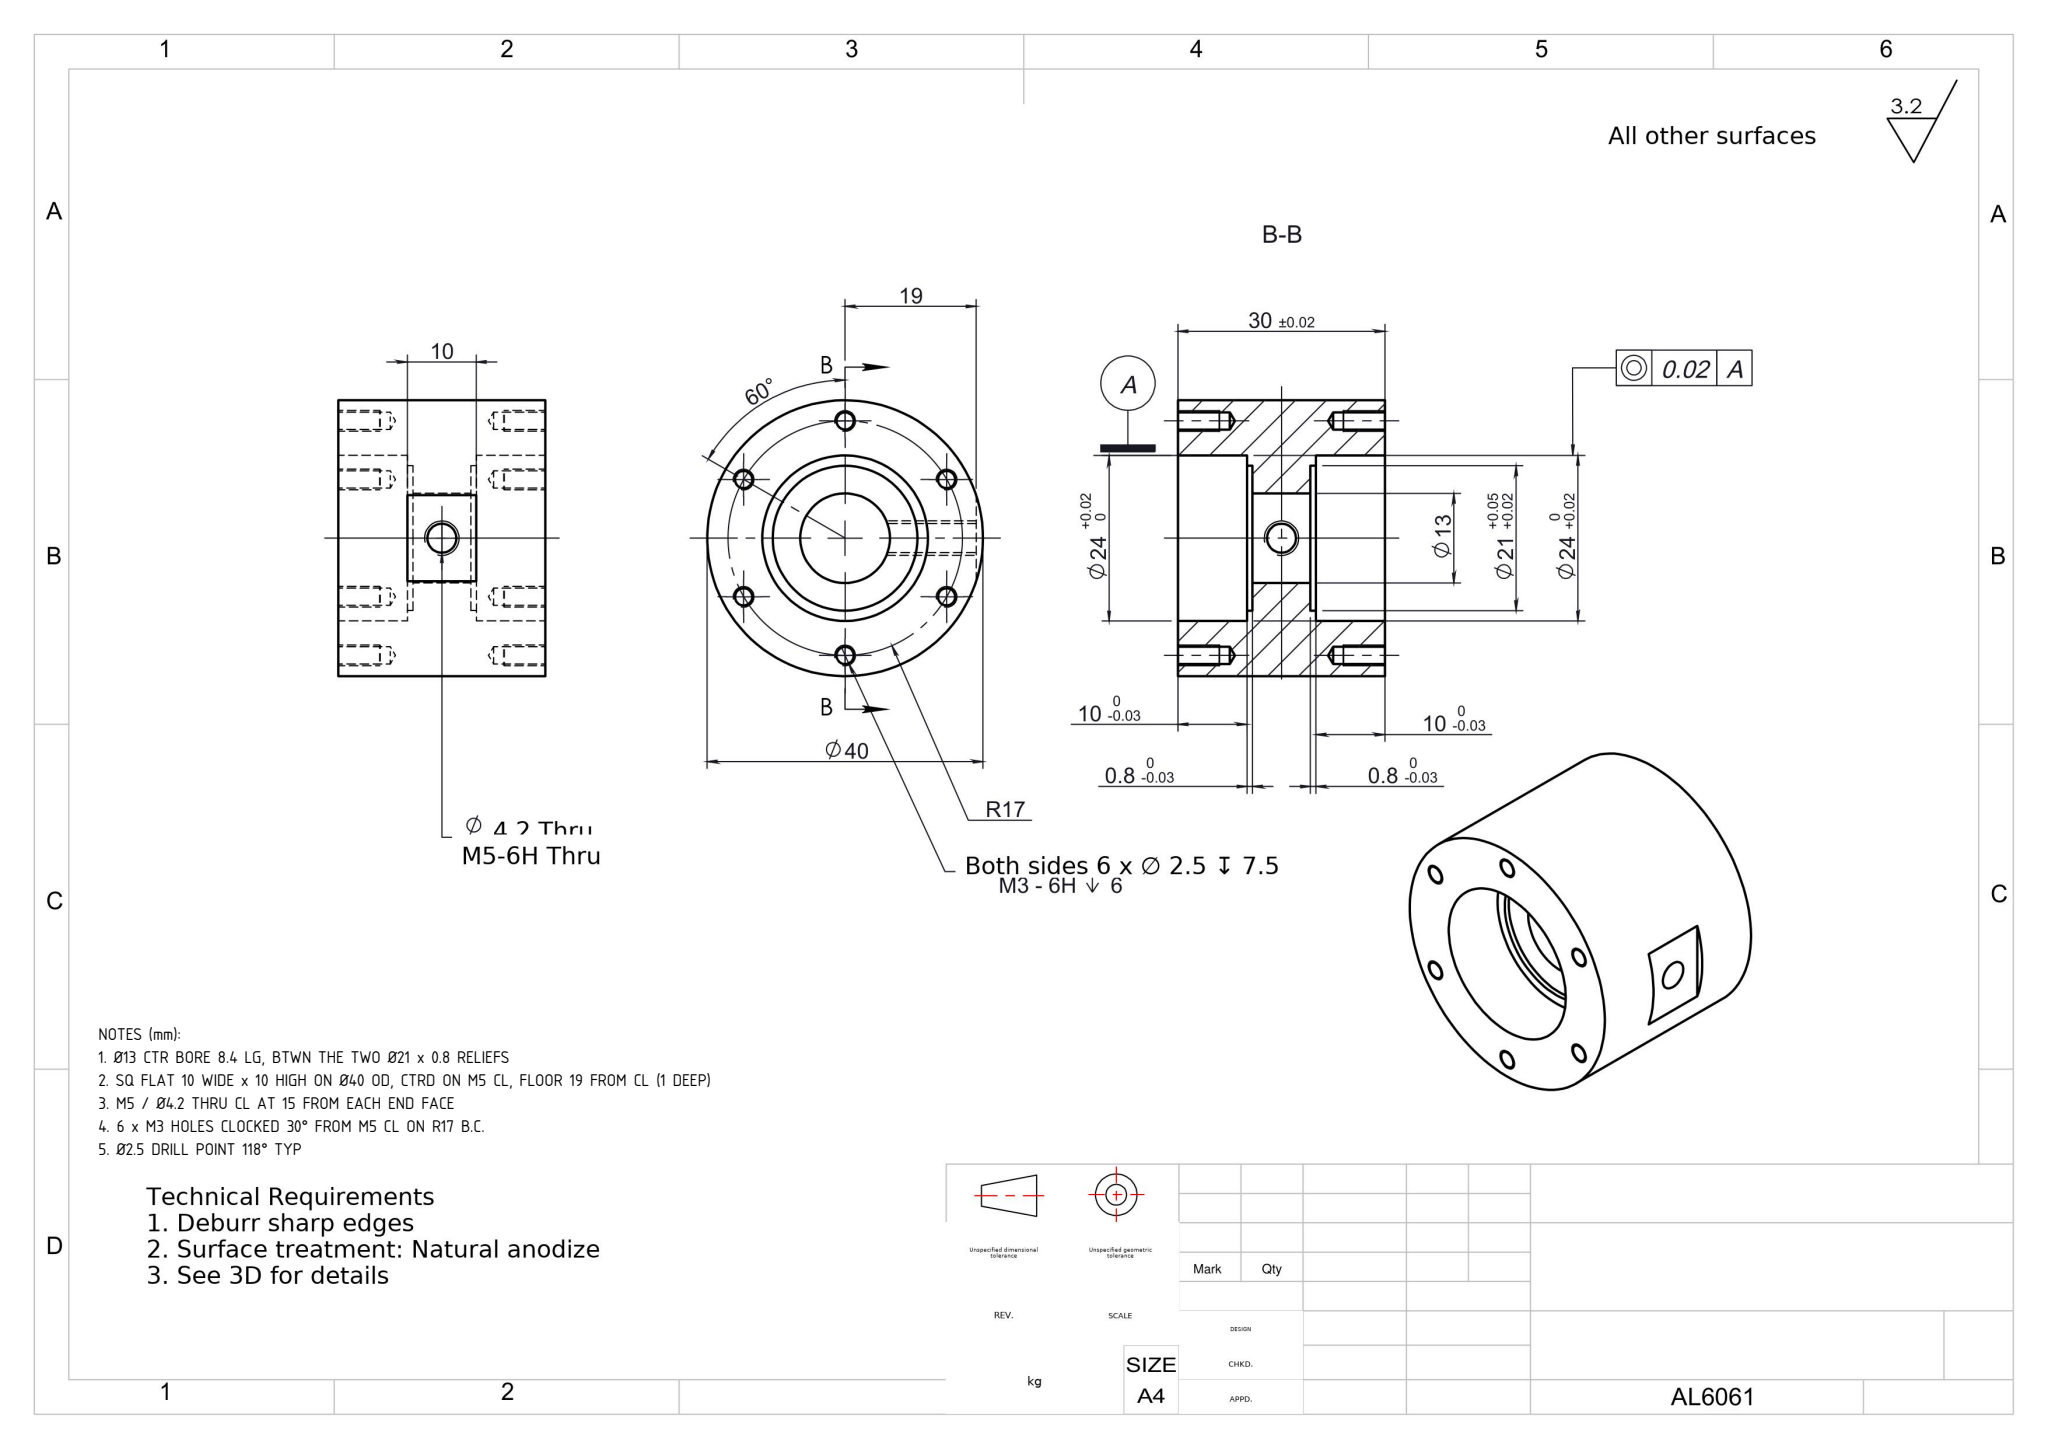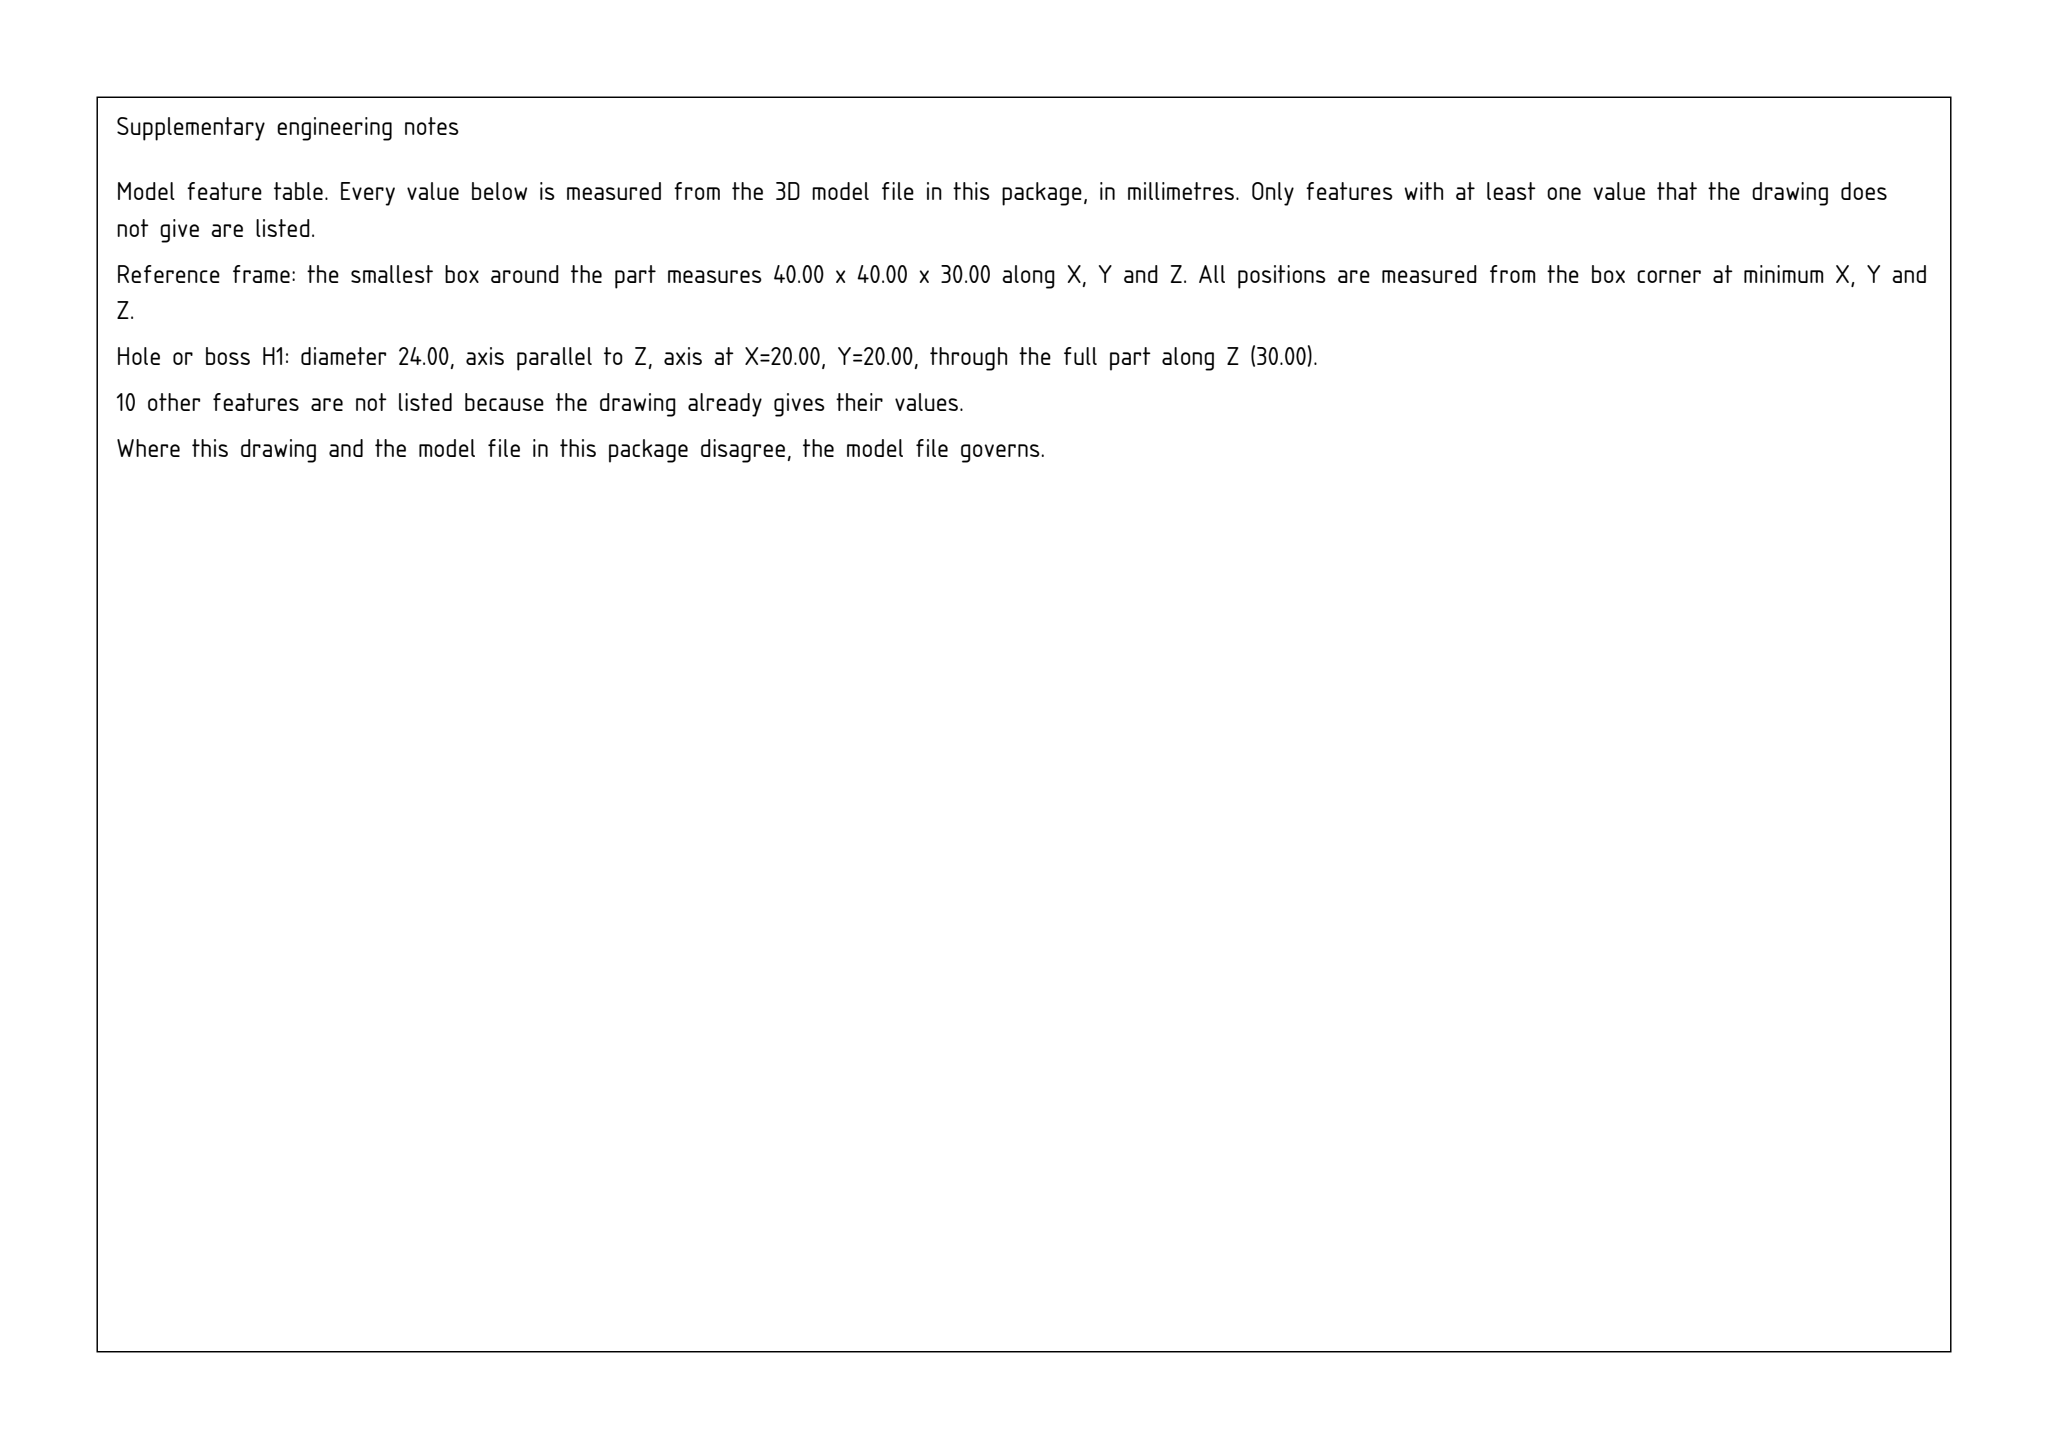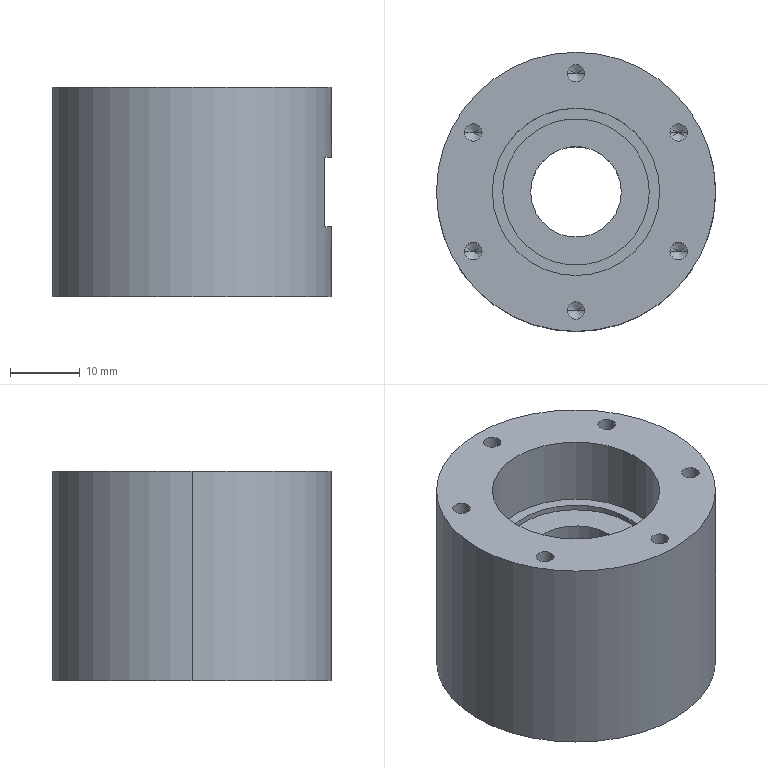Part | SolidWorks | mm | 1 solid | 71 faces | box 40 x 40 x 30 mm | volume 26268 mm3 | cylinder 38 | cone 24 | plane 9 | commonest cylinder face diameters 2.5 x24 21 x4 24 x4 4.2 x2 40 x2 13 x2
Drawing notes:
Ø13 CTR BORE 8.4 LG, BTWN THE TWO Ø21 x 0.8 RELIEFS | from the solid: cyl Ø13 axis z at (20,20) length 8.4; Ø21 x 0.8 reliefs bounded by planes z=10.8 and z=19.2
SQ FLAT 10 WIDE x 10 HIGH ON Ø40 OD, CTRD ON M5 CL, FLOOR 19 FROM CL (1 DEEP) | from the solid: plane normal X at x=39 (19 from Ø40 axis at x=20, 1 deep), spans z=10 to z=20, symmetric about y=20
M5 / Ø4.2 THRU CL AT 15 FROM EACH END FACE | from the solid: Ø4.2 cyl axis along X at y=20, z=15 = mid of 30 overall length
6 x M3 HOLES CLOCKED 30° FROM M5 CL ON R17 B.C. | from the solid: Ø2.5 holes at (20,3),(20,37),(5.28,11.5),(5.28,28.5),(34.72,11.5),(34.72,28.5) = 30°,90°,150°,210°,270°,330° about ctr (20,20); M5 axis at 0°
Ø2.5 DRILL POINT 118° TYP | from the solid: cones: included angle 118.0 on Ø2.5 holes
build123d program:
from build123d import *

# Parameters (mm, degrees)
SKETCH1_R             = 20
BOSS_EXTRUDE1_DEPTH   = 15
SKETCH2_R             = 6.5
CUT_EXTRUDE1_DEPTH    = 42.231
SKETCH3_R             = 12
CUT_EXTRUDE2_DEPTH    = 10
SKETCH4_R             = 10.5
CUT_EXTRUDE3_DEPTH    = 0.8
SKETCH6_W             = 2.1
SKETCH6_H             = 20
M3_TAPPED_HOLE1_D     = 2.5
M3_TAPPED_HOLE1_DEPTH = 7.5
M3_TAPPED_HOLE1_TIP   = 0.7511
M3_TAPPED_HOLE2_D     = 2.5
M3_TAPPED_HOLE2_DEPTH = 7.5
M3_TAPPED_HOLE2_TIP   = 0.7511
SKETCH11_W            = 1
SKETCH11_H            = 10
CUT_EXTRUDE4_DEPTH    = 26.5


with BuildPart() as part:
    # Sketch1 → Boss-Extrude1 (new, symmetric)
    with BuildSketch(Plane.XY):
        Circle(SKETCH1_R)
    extrude(amount=BOSS_EXTRUDE1_DEPTH, both=True)

    # Sketch2 → Cut-Extrude1 (cut, through all)
    with BuildSketch(Plane.XY.offset(15)):
        Circle(SKETCH2_R)
    extrude(amount=-CUT_EXTRUDE1_DEPTH, mode=Mode.SUBTRACT)

    # Sketch3 → Cut-Extrude2 (cut)
    with BuildSketch(Plane.XY.offset(15)):
        Circle(SKETCH3_R)
    cut_extrude2 = extrude(amount=-CUT_EXTRUDE2_DEPTH, mode=Mode.SUBTRACT)

    # Sketch4 → Cut-Extrude3 (cut)
    with BuildSketch(Plane.XY.offset(5)):
        Circle(SKETCH4_R)
    cut_extrude3 = extrude(amount=-CUT_EXTRUDE3_DEPTH, mode=Mode.SUBTRACT)

    # Mirror1: Cut-Extrude2, Cut-Extrude3 across plane
    add(cut_extrude2.mirror(Plane.XY), mode=Mode.SUBTRACT)
    add(cut_extrude3.mirror(Plane.XY), mode=Mode.SUBTRACT)

    # Sketch6 → M5 Tapped Hole1 (revolve, cut)
    with BuildSketch(Plane.ZX):
        with Locations((1.05, 10)):
            Rectangle(SKETCH6_W, SKETCH6_H)
    revolve(axis=Axis((-6.35, 0, 0), (1, 0, 0)), mode=Mode.SUBTRACT)

    # M3 Tapped Hole1
    with Locations(Plane(origin=(0, 0, -15), x_dir=(-1, 0, 0), z_dir=(0, 0, -1))):
        with Locations((0, 17), (14.722, 8.5), (14.722, -8.5), (0, -17), (-14.722, -8.5), (-14.722, 8.5)):
            Hole(M3_TAPPED_HOLE1_D / 2, depth=M3_TAPPED_HOLE1_DEPTH)
            with Locations((0, 0, -(M3_TAPPED_HOLE1_DEPTH + M3_TAPPED_HOLE1_TIP / 2))):  # 118° drill point
                Cone(0, M3_TAPPED_HOLE1_D / 2, M3_TAPPED_HOLE1_TIP, mode=Mode.SUBTRACT)

    # M3 Tapped Hole2
    with Locations(Plane.XY.offset(15)):
        with Locations((0, 17), (14.722, 8.5), (14.722, -8.5), (0, -17), (-14.722, -8.5), (-14.722, 8.5)):
            Hole(M3_TAPPED_HOLE2_D / 2, depth=M3_TAPPED_HOLE2_DEPTH)
            with Locations((0, 0, -(M3_TAPPED_HOLE2_DEPTH + M3_TAPPED_HOLE2_TIP / 2))):  # 118° drill point
                Cone(0, M3_TAPPED_HOLE2_D / 2, M3_TAPPED_HOLE2_TIP, mode=Mode.SUBTRACT)

    # Sketch11 → Cut-Extrude4 (cut, symmetric)
    with BuildSketch(Plane(origin=(0, 0, 0), x_dir=(1, 0, 0), z_dir=(0, 1, 0))):
        with Locations((19.5, 0)):
            Rectangle(SKETCH11_W, SKETCH11_H)
    extrude(amount=CUT_EXTRUDE4_DEPTH, both=True, mode=Mode.SUBTRACT)


solid = part.part